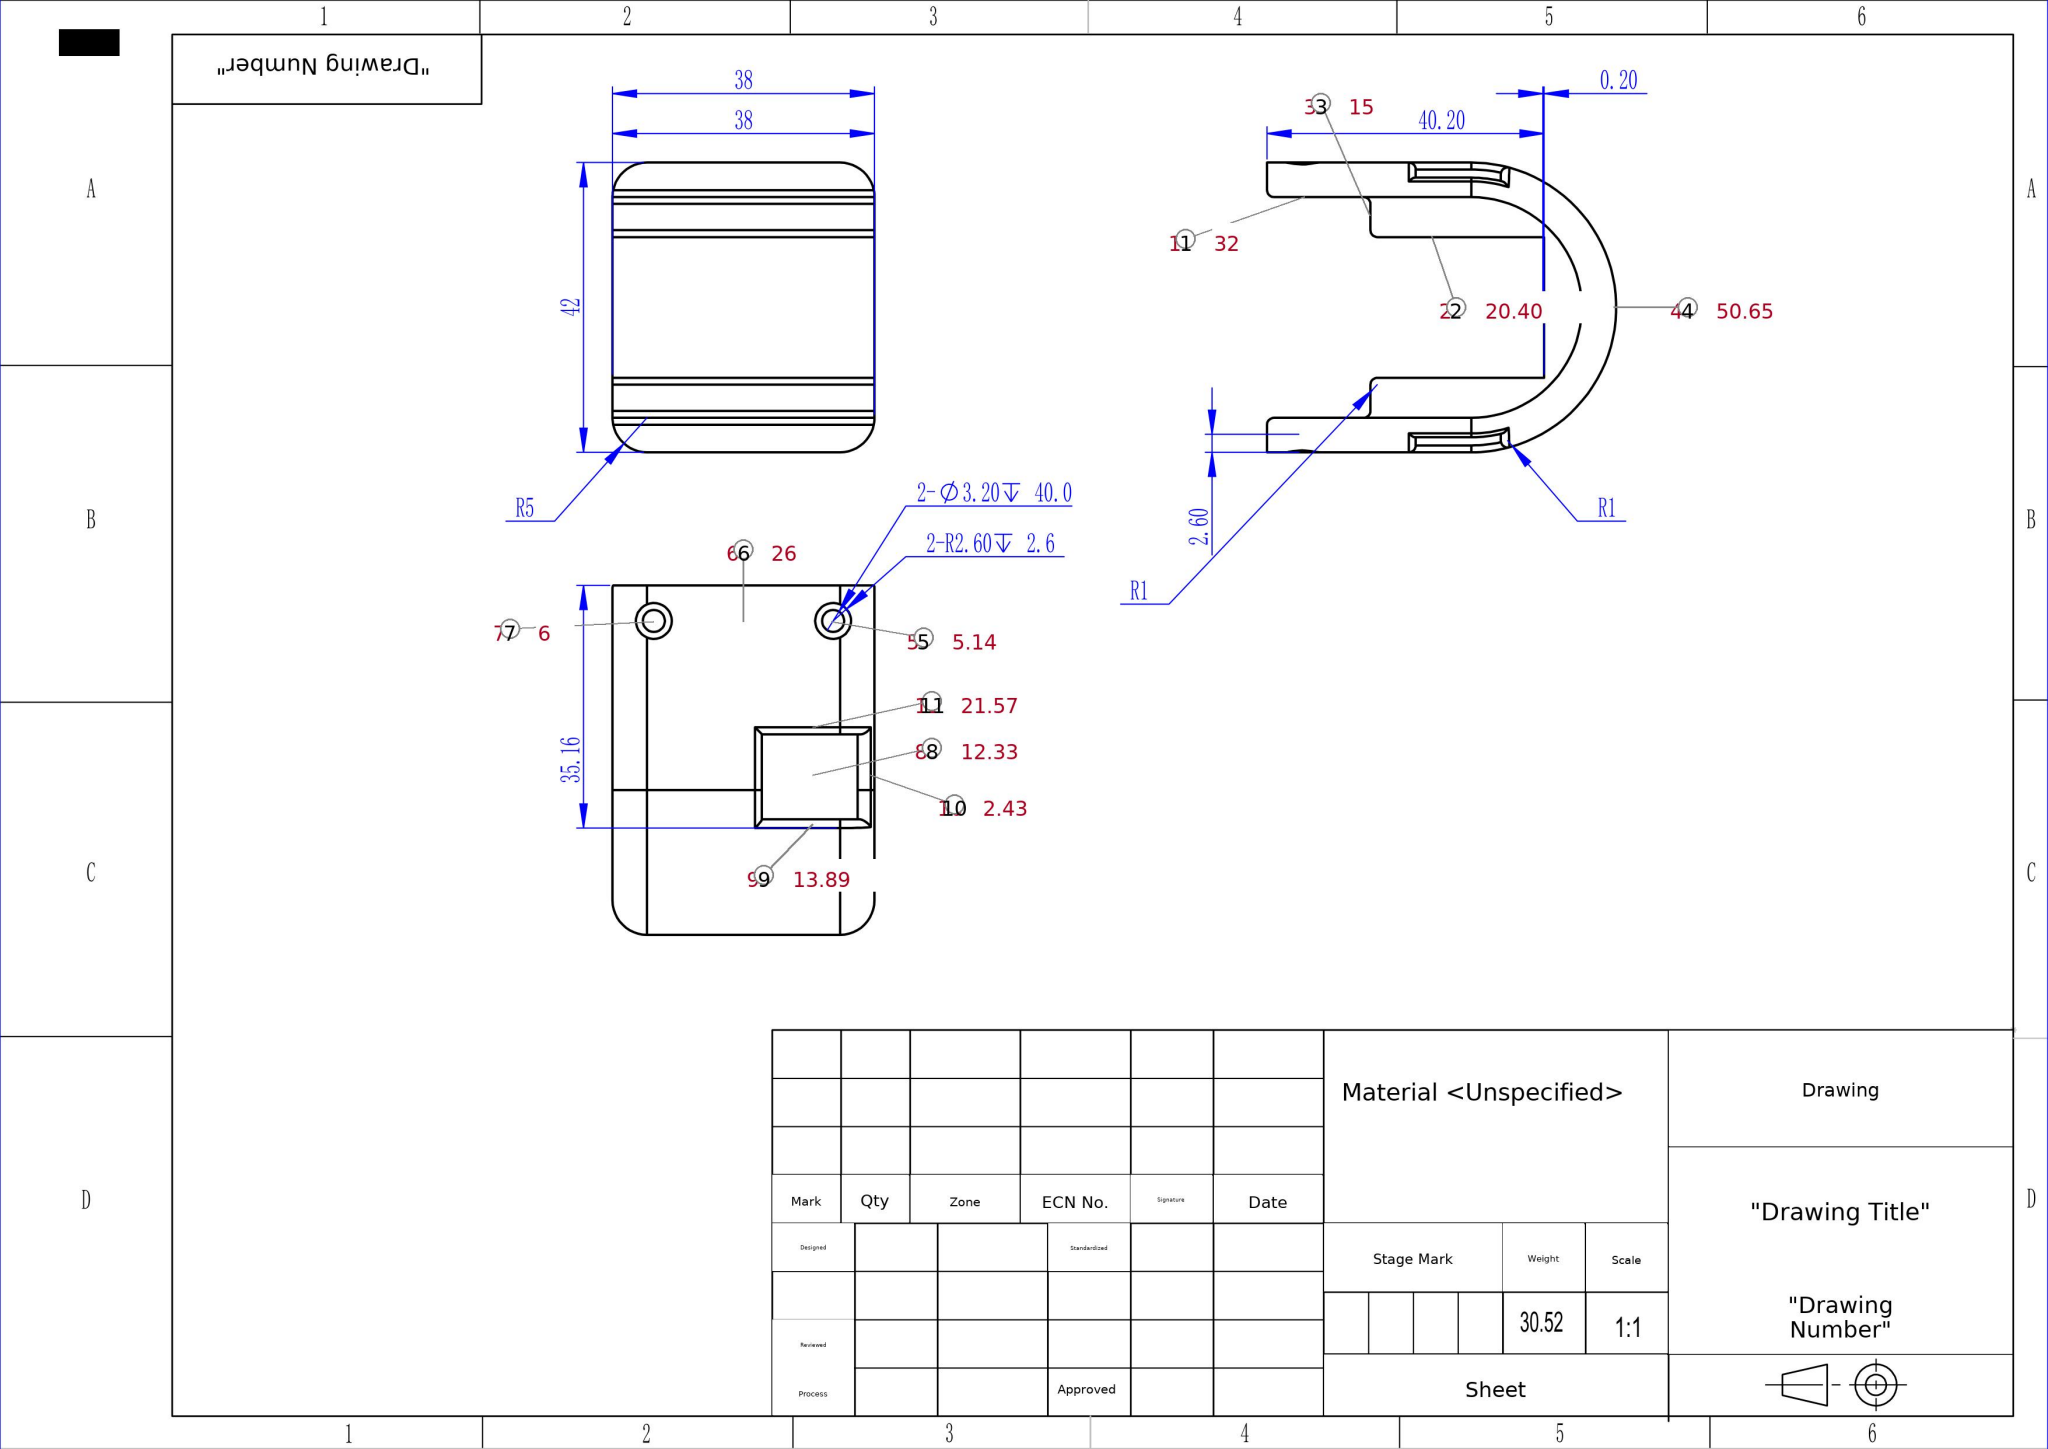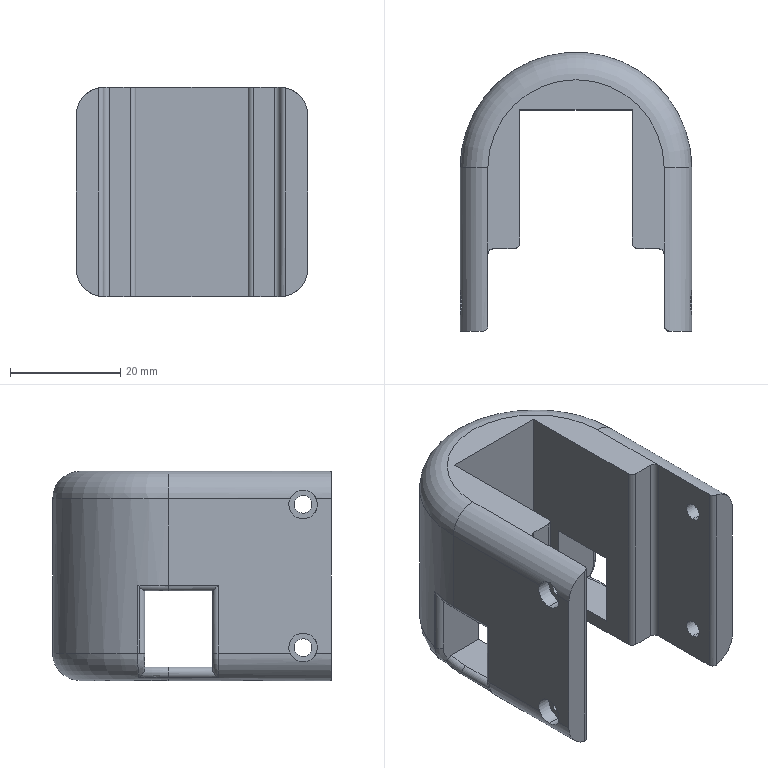Part | SolidWorks | mm | 1 solid | 71 faces | box 42 x 50.65 x 38 mm | volume 30518 mm3 | cylinder 36 | plane 25 | torus 8 | spline 2 | commonest cylinder face diameters 2 x15 5.2 x8 3.2 x8 10 x4 42 x1